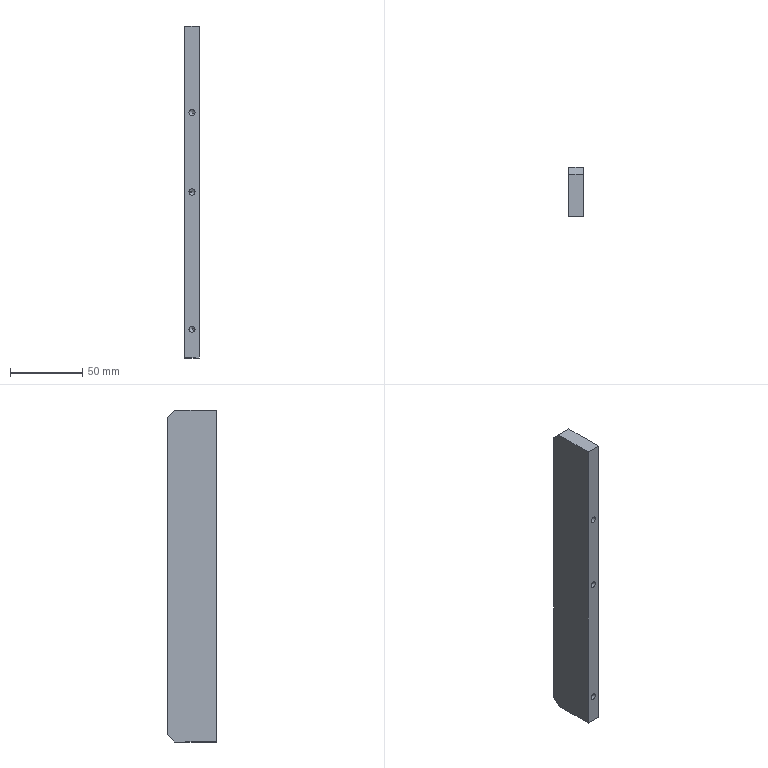Component | SolidWorks | 009-1 | 1 solid | 20 faces | box 10 x 34 x 230 mm | volume 77417 mm3 | plane 8 | cylinder 6 | cone 6 | commonest cylinder face diameters 4.2 x6 | material AL6061
build123d program:
from build123d import *

# Parameters (mm, degrees)
BOSS_EXTRUDE1_DEPTH   = 10
M5_TAPPED_HOLE2_D     = 4.2
M5_TAPPED_HOLE2_DEPTH = 12.4
M5_TAPPED_HOLE2_TIP   = 1.262
CHAMFER1_SIZE         = 5


with BuildPart() as part:
    # Sketch1 → Boss-Extrude1 (new body)
    with BuildSketch(Plane.XY):
        Polygon((0, 0), (0, 34), (10, 34), (230, 34), (230, 0), align=None)
    extrude(amount=BOSS_EXTRUDE1_DEPTH)

    # M5 Tapped Hole2
    with Locations(Plane(origin=(0, 0, 0), x_dir=(-1, 0, 0), z_dir=(0, -1, 0))):
        with Locations((-60, -5), (-115, -5), (-210, -5)):
            Hole(M5_TAPPED_HOLE2_D / 2, depth=M5_TAPPED_HOLE2_DEPTH)
            with Locations((0, 0, -(M5_TAPPED_HOLE2_DEPTH + M5_TAPPED_HOLE2_TIP / 2))):  # 118° drill point
                Cone(0, M5_TAPPED_HOLE2_D / 2, M5_TAPPED_HOLE2_TIP, mode=Mode.SUBTRACT)

    # Chamfer1
    chamfer1_edges = [part.edges().sort_by_distance(p)[0] for p in [
        (0, 34, 5),
        (230, 34, 5),
    ]]
    chamfer(chamfer1_edges, length=CHAMFER1_SIZE)


solid = part.part

# Placed as in the assembly
solid = solid.moved(Location((-210.455, -145.942, -128.376), (0, 90, 0)))